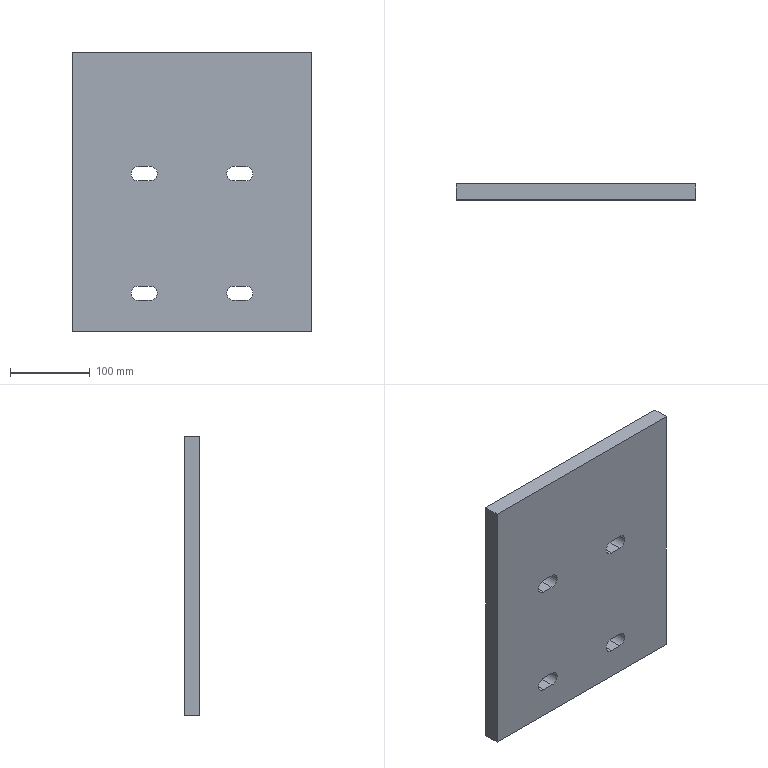Component | SolidWorks | WeldedI-beam-1_250I-beamMountingPlate-1 | 1 solid | 22 faces | box 300 x 20 x 350 mm | volume 2058042 mm3 | plane 14 | cylinder 8 | commonest cylinder face diameters 18 x8 | material Plain Carbon Steel
STEP:
#1=CARTESIAN_POINT('',(-256.79,105.58,213.545));
#2=VERTEX_POINT('',#1);
#3=CARTESIAN_POINT('',(-256.79,105.58,227.325));
#4=VERTEX_POINT('',#3);
#5=CARTESIAN_POINT('',(-256.79,105.58,213.545));
#6=DIRECTION('',(0.,0.,1.));
#7=VECTOR('',#6,39.37);
#8=LINE('',#5,#7);
#9=EDGE_CURVE('',#2,#4,#8,.T.);
#10=ORIENTED_EDGE('',*,*,#9,.F.);
#11=CARTESIAN_POINT('',(-256.79,104.793,213.545));
#12=VERTEX_POINT('',#11);
#13=CARTESIAN_POINT('',(-256.79,104.793,213.545));
#14=DIRECTION('',(0.,1.,0.));
#15=VECTOR('',#14,39.37);
#16=LINE('',#13,#15);
#17=EDGE_CURVE('',#12,#2,#16,.T.);
#18=ORIENTED_EDGE('',*,*,#17,.F.);
#19=CARTESIAN_POINT('',(-256.79,104.793,227.325));
#20=VERTEX_POINT('',#19);
#21=CARTESIAN_POINT('',(-256.79,104.793,213.545));
#22=DIRECTION('',(0.,0.,1.));
#23=VECTOR('',#22,39.37);
#24=LINE('',#21,#23);
#25=EDGE_CURVE('',#12,#20,#24,.T.);
#26=ORIENTED_EDGE('',*,*,#25,.T.);
#27=CARTESIAN_POINT('',(-256.79,104.793,227.325));
#28=DIRECTION('',(0.,1.,0.));
#29=VECTOR('',#28,39.37);
#30=LINE('',#27,#29);
#31=EDGE_CURVE('',#20,#4,#30,.T.);
#32=ORIENTED_EDGE('',*,*,#31,.T.);
#33=EDGE_LOOP('',(#10,#18,#26,#32));
#34=FACE_OUTER_BOUND('',#33,.T.);
#35=CARTESIAN_POINT('',(-256.79,104.793,213.545));
#36=DIRECTION('',(-1.,0.,0.));
#37=DIRECTION('',(0.,0.,1.));
#38=AXIS2_PLACEMENT_3D('',#35,#36,#37);
#39=PLANE('',#38);
#40=ADVANCED_FACE('',(#34),#39,.T.);
#41=CARTESIAN_POINT('',(-244.979,105.58,213.545));
#42=VERTEX_POINT('',#41);
#43=CARTESIAN_POINT('',(-256.79,105.58,213.545));
#44=DIRECTION('',(-1.,0.,0.));
#45=VECTOR('',#44,39.37);
#46=LINE('',#43,#45);
#47=EDGE_CURVE('',#42,#2,#46,.T.);
#48=ORIENTED_EDGE('',*,*,#47,.F.);
#49=CARTESIAN_POINT('',(-244.979,104.793,213.545));
#50=VERTEX_POINT('',#49);
#51=CARTESIAN_POINT('',(-244.979,104.793,213.545));
#52=DIRECTION('',(0.,1.,0.));
#53=VECTOR('',#52,39.37);
#54=LINE('',#51,#53);
#55=EDGE_CURVE('',#50,#42,#54,.T.);
#56=ORIENTED_EDGE('',*,*,#55,.F.);
#57=CARTESIAN_POINT('',(-256.79,104.793,213.545));
#58=DIRECTION('',(-1.,0.,0.));
#59=VECTOR('',#58,39.37);
#60=LINE('',#57,#59);
#61=EDGE_CURVE('',#50,#12,#60,.T.);
#62=ORIENTED_EDGE('',*,*,#61,.T.);
#63=ORIENTED_EDGE('',*,*,#17,.T.);
#64=EDGE_LOOP('',(#48,#56,#62,#63));
#65=FACE_OUTER_BOUND('',#64,.T.);
#66=CARTESIAN_POINT('',(-256.79,104.793,213.545));
#67=DIRECTION('',(0.,0.,-1.));
#68=DIRECTION('',(-1.,0.,0.));
#69=AXIS2_PLACEMENT_3D('',#66,#67,#68);
#70=PLANE('',#69);
#71=ADVANCED_FACE('',(#65),#70,.T.);
#72=CARTESIAN_POINT('',(-244.979,105.58,227.325));
#73=VERTEX_POINT('',#72);
#74=CARTESIAN_POINT('',(-244.979,105.58,213.545));
#75=DIRECTION('',(-0.,0.,-1.));
#76=VECTOR('',#75,39.37);
#77=LINE('',#74,#76);
#78=EDGE_CURVE('',#73,#42,#77,.T.);
#79=ORIENTED_EDGE('',*,*,#78,.F.);
#80=CARTESIAN_POINT('',(-244.979,104.793,227.325));
#81=VERTEX_POINT('',#80);
#82=CARTESIAN_POINT('',(-244.979,104.793,227.325));
#83=DIRECTION('',(0.,1.,0.));
#84=VECTOR('',#83,39.37);
#85=LINE('',#82,#84);
#86=EDGE_CURVE('',#81,#73,#85,.T.);
#87=ORIENTED_EDGE('',*,*,#86,.F.);
#88=CARTESIAN_POINT('',(-244.979,104.793,213.545));
#89=DIRECTION('',(-0.,0.,-1.));
#90=VECTOR('',#89,39.37);
#91=LINE('',#88,#90);
#92=EDGE_CURVE('',#81,#50,#91,.T.);
#93=ORIENTED_EDGE('',*,*,#92,.T.);
#94=ORIENTED_EDGE('',*,*,#55,.T.);
#95=EDGE_LOOP('',(#79,#87,#93,#94));
#96=FACE_OUTER_BOUND('',#95,.T.);
#97=CARTESIAN_POINT('',(-244.979,104.793,213.545));
#98=DIRECTION('',(1.,0.,-0.));
#99=DIRECTION('',(-0.,0.,-1.));
#100=AXIS2_PLACEMENT_3D('',#97,#98,#99);
#101=PLANE('',#100);
#102=ADVANCED_FACE('',(#96),#101,.T.);
#103=CARTESIAN_POINT('',(-256.79,105.58,227.325));
#104=DIRECTION('',(1.,0.,0.));
#105=VECTOR('',#104,39.37);
#106=LINE('',#103,#105);
#107=EDGE_CURVE('',#4,#73,#106,.T.);
#108=ORIENTED_EDGE('',*,*,#107,.F.);
#109=ORIENTED_EDGE('',*,*,#31,.F.);
#110=CARTESIAN_POINT('',(-256.79,104.793,227.325));
#111=DIRECTION('',(1.,0.,0.));
#112=VECTOR('',#111,39.37);
#113=LINE('',#110,#112);
#114=EDGE_CURVE('',#20,#81,#113,.T.);
#115=ORIENTED_EDGE('',*,*,#114,.T.);
#116=ORIENTED_EDGE('',*,*,#86,.T.);
#117=EDGE_LOOP('',(#108,#109,#115,#116));
#118=FACE_OUTER_BOUND('',#117,.T.);
#119=CARTESIAN_POINT('',(-256.79,104.793,227.325));
#120=DIRECTION('',(0.,0.,1.));
#121=DIRECTION('',(1.,0.,0.));
#122=AXIS2_PLACEMENT_3D('',#119,#120,#121);
#123=PLANE('',#122);
#124=ADVANCED_FACE('',(#118),#123,.T.);
#125=CARTESIAN_POINT('',(-252.951,104.793,220.986));
#126=VERTEX_POINT('',#125);
#127=CARTESIAN_POINT('',(-253.542,104.793,220.986));
#128=VERTEX_POINT('',#127);
#129=CARTESIAN_POINT('',(-253.542,104.793,220.986));
#130=DIRECTION('',(-1.,0.,0.));
#131=VECTOR('',#130,39.37);
#132=LINE('',#129,#131);
#133=EDGE_CURVE('',#126,#128,#132,.T.);
#134=ORIENTED_EDGE('',*,*,#133,.T.);
#135=CARTESIAN_POINT('',(-253.542,104.793,221.695));
#136=VERTEX_POINT('',#135);
#137=CARTESIAN_POINT('',(-253.542,104.793,221.34));
#138=DIRECTION('',(0.,1.,0.));
#139=DIRECTION('',(0.,0.,1.));
#140=AXIS2_PLACEMENT_3D('',#137,#138,#139);
#141=CIRCLE('',#140,0.3543);
#142=EDGE_CURVE('',#128,#136,#141,.T.);
#143=ORIENTED_EDGE('',*,*,#142,.T.);
#144=CARTESIAN_POINT('',(-252.951,104.793,221.695));
#145=VERTEX_POINT('',#144);
#146=CARTESIAN_POINT('',(-253.542,104.793,221.695));
#147=DIRECTION('',(1.,0.,0.));
#148=VECTOR('',#147,39.37);
#149=LINE('',#146,#148);
#150=EDGE_CURVE('',#136,#145,#149,.T.);
#151=ORIENTED_EDGE('',*,*,#150,.T.);
#152=CARTESIAN_POINT('',(-252.951,104.793,221.34));
#153=DIRECTION('',(0.,1.,0.));
#154=DIRECTION('',(0.,0.,1.));
#155=AXIS2_PLACEMENT_3D('',#152,#153,#154);
#156=CIRCLE('',#155,0.3543);
#157=EDGE_CURVE('',#145,#126,#156,.T.);
#158=ORIENTED_EDGE('',*,*,#157,.T.);
#159=EDGE_LOOP('',(#134,#143,#151,#158));
#160=FACE_BOUND('',#159,.T.);
#161=CARTESIAN_POINT('',(-248.227,104.793,220.986));
#162=VERTEX_POINT('',#161);
#163=CARTESIAN_POINT('',(-248.818,104.793,220.986));
#164=VERTEX_POINT('',#163);
#165=CARTESIAN_POINT('',(-248.818,104.793,220.986));
#166=DIRECTION('',(-1.,0.,-0.));
#167=VECTOR('',#166,39.37);
#168=LINE('',#165,#167);
#169=EDGE_CURVE('',#162,#164,#168,.T.);
#170=ORIENTED_EDGE('',*,*,#169,.T.);
#171=CARTESIAN_POINT('',(-248.818,104.793,221.695));
#172=VERTEX_POINT('',#171);
#173=CARTESIAN_POINT('',(-248.818,104.793,221.34));
#174=DIRECTION('',(0.,1.,0.));
#175=DIRECTION('',(0.,0.,1.));
#176=AXIS2_PLACEMENT_3D('',#173,#174,#175);
#177=CIRCLE('',#176,0.3543);
#178=EDGE_CURVE('',#164,#172,#177,.T.);
#179=ORIENTED_EDGE('',*,*,#178,.T.);
#180=CARTESIAN_POINT('',(-248.227,104.793,221.695));
#181=VERTEX_POINT('',#180);
#182=CARTESIAN_POINT('',(-248.818,104.793,221.695));
#183=DIRECTION('',(1.,0.,-0.));
#184=VECTOR('',#183,39.37);
#185=LINE('',#182,#184);
#186=EDGE_CURVE('',#172,#181,#185,.T.);
#187=ORIENTED_EDGE('',*,*,#186,.T.);
#188=CARTESIAN_POINT('',(-248.227,104.793,221.34));
#189=DIRECTION('',(0.,1.,0.));
#190=DIRECTION('',(0.,0.,1.));
#191=AXIS2_PLACEMENT_3D('',#188,#189,#190);
#192=CIRCLE('',#191,0.3543);
#193=EDGE_CURVE('',#181,#162,#192,.T.);
#194=ORIENTED_EDGE('',*,*,#193,.T.);
#195=EDGE_LOOP('',(#170,#179,#187,#194));
#196=FACE_BOUND('',#195,.T.);
#197=CARTESIAN_POINT('',(-252.951,104.793,215.08));
#198=VERTEX_POINT('',#197);
#199=CARTESIAN_POINT('',(-253.542,104.793,215.08));
#200=VERTEX_POINT('',#199);
#201=CARTESIAN_POINT('',(-253.542,104.793,215.08));
#202=DIRECTION('',(-1.,0.,0.));
#203=VECTOR('',#202,39.37);
#204=LINE('',#201,#203);
#205=EDGE_CURVE('',#198,#200,#204,.T.);
#206=ORIENTED_EDGE('',*,*,#205,.T.);
#207=CARTESIAN_POINT('',(-253.542,104.793,215.789));
#208=VERTEX_POINT('',#207);
#209=CARTESIAN_POINT('',(-253.542,104.793,215.435));
#210=DIRECTION('',(0.,1.,0.));
#211=DIRECTION('',(0.,0.,1.));
#212=AXIS2_PLACEMENT_3D('',#209,#210,#211);
#213=CIRCLE('',#212,0.3543);
#214=EDGE_CURVE('',#200,#208,#213,.T.);
#215=ORIENTED_EDGE('',*,*,#214,.T.);
#216=CARTESIAN_POINT('',(-252.951,104.793,215.789));
#217=VERTEX_POINT('',#216);
#218=CARTESIAN_POINT('',(-253.542,104.793,215.789));
#219=DIRECTION('',(1.,0.,0.));
#220=VECTOR('',#219,39.37);
#221=LINE('',#218,#220);
#222=EDGE_CURVE('',#208,#217,#221,.T.);
#223=ORIENTED_EDGE('',*,*,#222,.T.);
#224=CARTESIAN_POINT('',(-252.951,104.793,215.435));
#225=DIRECTION('',(0.,1.,0.));
#226=DIRECTION('',(0.,0.,1.));
#227=AXIS2_PLACEMENT_3D('',#224,#225,#226);
#228=CIRCLE('',#227,0.3543);
#229=EDGE_CURVE('',#217,#198,#228,.T.);
#230=ORIENTED_EDGE('',*,*,#229,.T.);
#231=EDGE_LOOP('',(#206,#215,#223,#230));
#232=FACE_BOUND('',#231,.T.);
#233=CARTESIAN_POINT('',(-248.227,104.793,215.08));
#234=VERTEX_POINT('',#233);
#235=CARTESIAN_POINT('',(-248.818,104.793,215.08));
#236=VERTEX_POINT('',#235);
#237=CARTESIAN_POINT('',(-248.818,104.793,215.08));
#238=DIRECTION('',(-1.,0.,0.));
#239=VECTOR('',#238,39.37);
#240=LINE('',#237,#239);
#241=EDGE_CURVE('',#234,#236,#240,.T.);
#242=ORIENTED_EDGE('',*,*,#241,.T.);
#243=CARTESIAN_POINT('',(-248.818,104.793,215.789));
#244=VERTEX_POINT('',#243);
#245=CARTESIAN_POINT('',(-248.818,104.793,215.435));
#246=DIRECTION('',(0.,1.,0.));
#247=DIRECTION('',(0.,0.,1.));
#248=AXIS2_PLACEMENT_3D('',#245,#246,#247);
#249=CIRCLE('',#248,0.3543);
#250=EDGE_CURVE('',#236,#244,#249,.T.);
#251=ORIENTED_EDGE('',*,*,#250,.T.);
#252=CARTESIAN_POINT('',(-248.227,104.793,215.789));
#253=VERTEX_POINT('',#252);
#254=CARTESIAN_POINT('',(-248.818,104.793,215.789));
#255=DIRECTION('',(1.,0.,0.));
#256=VECTOR('',#255,39.37);
#257=LINE('',#254,#256);
#258=EDGE_CURVE('',#244,#253,#257,.T.);
#259=ORIENTED_EDGE('',*,*,#258,.T.);
#260=CARTESIAN_POINT('',(-248.227,104.793,215.435));
#261=DIRECTION('',(0.,1.,0.));
#262=DIRECTION('',(0.,0.,1.));
#263=AXIS2_PLACEMENT_3D('',#260,#261,#262);
#264=CIRCLE('',#263,0.3543);
#265=EDGE_CURVE('',#253,#234,#264,.T.);
#266=ORIENTED_EDGE('',*,*,#265,.T.);
#267=EDGE_LOOP('',(#242,#251,#259,#266));
#268=FACE_BOUND('',#267,.T.);
#269=ORIENTED_EDGE('',*,*,#25,.F.);
#270=ORIENTED_EDGE('',*,*,#61,.F.);
#271=ORIENTED_EDGE('',*,*,#92,.F.);
#272=ORIENTED_EDGE('',*,*,#114,.F.);
#273=EDGE_LOOP('',(#269,#270,#271,#272));
#274=FACE_OUTER_BOUND('',#273,.T.);
#275=CARTESIAN_POINT('',(-256.79,104.793,213.545));
#276=DIRECTION('',(0.,1.,0.));
#277=DIRECTION('',(0.,0.,1.));
#278=AXIS2_PLACEMENT_3D('',#275,#276,#277);
#279=PLANE('',#278);
#280=ADVANCED_FACE('',(#160,#196,#232,#268,#274),#279,.F.);
#281=CARTESIAN_POINT('',(-253.542,105.58,220.986));
#282=VERTEX_POINT('',#281);
#283=CARTESIAN_POINT('',(-253.542,105.58,221.695));
#284=VERTEX_POINT('',#283);
#285=CARTESIAN_POINT('',(-253.542,105.58,221.34));
#286=DIRECTION('',(0.,1.,0.));
#287=DIRECTION('',(0.,0.,1.));
#288=AXIS2_PLACEMENT_3D('',#285,#286,#287);
#289=CIRCLE('',#288,0.3543);
#290=EDGE_CURVE('',#282,#284,#289,.T.);
#291=ORIENTED_EDGE('',*,*,#290,.F.);
#292=CARTESIAN_POINT('',(-252.951,105.58,220.986));
#293=VERTEX_POINT('',#292);
#294=CARTESIAN_POINT('',(-253.542,105.58,220.986));
#295=DIRECTION('',(-1.,0.,0.));
#296=VECTOR('',#295,39.37);
#297=LINE('',#294,#296);
#298=EDGE_CURVE('',#293,#282,#297,.T.);
#299=ORIENTED_EDGE('',*,*,#298,.F.);
#300=CARTESIAN_POINT('',(-252.951,105.58,221.695));
#301=VERTEX_POINT('',#300);
#302=CARTESIAN_POINT('',(-252.951,105.58,221.34));
#303=DIRECTION('',(0.,1.,0.));
#304=DIRECTION('',(0.,0.,1.));
#305=AXIS2_PLACEMENT_3D('',#302,#303,#304);
#306=CIRCLE('',#305,0.3543);
#307=EDGE_CURVE('',#301,#293,#306,.T.);
#308=ORIENTED_EDGE('',*,*,#307,.F.);
#309=CARTESIAN_POINT('',(-253.542,105.58,221.695));
#310=DIRECTION('',(1.,0.,0.));
#311=VECTOR('',#310,39.37);
#312=LINE('',#309,#311);
#313=EDGE_CURVE('',#284,#301,#312,.T.);
#314=ORIENTED_EDGE('',*,*,#313,.F.);
#315=EDGE_LOOP('',(#291,#299,#308,#314));
#316=FACE_BOUND('',#315,.T.);
#317=CARTESIAN_POINT('',(-248.818,105.58,220.986));
#318=VERTEX_POINT('',#317);
#319=CARTESIAN_POINT('',(-248.818,105.58,221.695));
#320=VERTEX_POINT('',#319);
#321=CARTESIAN_POINT('',(-248.818,105.58,221.34));
#322=DIRECTION('',(0.,1.,0.));
#323=DIRECTION('',(0.,0.,1.));
#324=AXIS2_PLACEMENT_3D('',#321,#322,#323);
#325=CIRCLE('',#324,0.3543);
#326=EDGE_CURVE('',#318,#320,#325,.T.);
#327=ORIENTED_EDGE('',*,*,#326,.F.);
#328=CARTESIAN_POINT('',(-248.227,105.58,220.986));
#329=VERTEX_POINT('',#328);
#330=CARTESIAN_POINT('',(-248.818,105.58,220.986));
#331=DIRECTION('',(-1.,0.,-0.));
#332=VECTOR('',#331,39.37);
#333=LINE('',#330,#332);
#334=EDGE_CURVE('',#329,#318,#333,.T.);
#335=ORIENTED_EDGE('',*,*,#334,.F.);
#336=CARTESIAN_POINT('',(-248.227,105.58,221.695));
#337=VERTEX_POINT('',#336);
#338=CARTESIAN_POINT('',(-248.227,105.58,221.34));
#339=DIRECTION('',(0.,1.,0.));
#340=DIRECTION('',(0.,0.,1.));
#341=AXIS2_PLACEMENT_3D('',#338,#339,#340);
#342=CIRCLE('',#341,0.3543);
#343=EDGE_CURVE('',#337,#329,#342,.T.);
#344=ORIENTED_EDGE('',*,*,#343,.F.);
#345=CARTESIAN_POINT('',(-248.818,105.58,221.695));
#346=DIRECTION('',(1.,0.,-0.));
#347=VECTOR('',#346,39.37);
#348=LINE('',#345,#347);
#349=EDGE_CURVE('',#320,#337,#348,.T.);
#350=ORIENTED_EDGE('',*,*,#349,.F.);
#351=EDGE_LOOP('',(#327,#335,#344,#350));
#352=FACE_BOUND('',#351,.T.);
#353=CARTESIAN_POINT('',(-253.542,105.58,215.08));
#354=VERTEX_POINT('',#353);
#355=CARTESIAN_POINT('',(-253.542,105.58,215.789));
#356=VERTEX_POINT('',#355);
#357=CARTESIAN_POINT('',(-253.542,105.58,215.435));
#358=DIRECTION('',(0.,1.,0.));
#359=DIRECTION('',(0.,0.,1.));
#360=AXIS2_PLACEMENT_3D('',#357,#358,#359);
#361=CIRCLE('',#360,0.3543);
#362=EDGE_CURVE('',#354,#356,#361,.T.);
#363=ORIENTED_EDGE('',*,*,#362,.F.);
#364=CARTESIAN_POINT('',(-252.951,105.58,215.08));
#365=VERTEX_POINT('',#364);
#366=CARTESIAN_POINT('',(-253.542,105.58,215.08));
#367=DIRECTION('',(-1.,0.,0.));
#368=VECTOR('',#367,39.37);
#369=LINE('',#366,#368);
#370=EDGE_CURVE('',#365,#354,#369,.T.);
#371=ORIENTED_EDGE('',*,*,#370,.F.);
#372=CARTESIAN_POINT('',(-252.951,105.58,215.789));
#373=VERTEX_POINT('',#372);
#374=CARTESIAN_POINT('',(-252.951,105.58,215.435));
#375=DIRECTION('',(0.,1.,0.));
#376=DIRECTION('',(0.,0.,1.));
#377=AXIS2_PLACEMENT_3D('',#374,#375,#376);
#378=CIRCLE('',#377,0.3543);
#379=EDGE_CURVE('',#373,#365,#378,.T.);
#380=ORIENTED_EDGE('',*,*,#379,.F.);
#381=CARTESIAN_POINT('',(-253.542,105.58,215.789));
#382=DIRECTION('',(1.,0.,0.));
#383=VECTOR('',#382,39.37);
#384=LINE('',#381,#383);
#385=EDGE_CURVE('',#356,#373,#384,.T.);
#386=ORIENTED_EDGE('',*,*,#385,.F.);
#387=EDGE_LOOP('',(#363,#371,#380,#386));
#388=FACE_BOUND('',#387,.T.);
#389=CARTESIAN_POINT('',(-248.818,105.58,215.08));
#390=VERTEX_POINT('',#389);
#391=CARTESIAN_POINT('',(-248.818,105.58,215.789));
#392=VERTEX_POINT('',#391);
#393=CARTESIAN_POINT('',(-248.818,105.58,215.435));
#394=DIRECTION('',(0.,1.,0.));
#395=DIRECTION('',(0.,0.,1.));
#396=AXIS2_PLACEMENT_3D('',#393,#394,#395);
#397=CIRCLE('',#396,0.3543);
#398=EDGE_CURVE('',#390,#392,#397,.T.);
#399=ORIENTED_EDGE('',*,*,#398,.F.);
#400=CARTESIAN_POINT('',(-248.227,105.58,215.08));
#401=VERTEX_POINT('',#400);
#402=CARTESIAN_POINT('',(-248.818,105.58,215.08));
#403=DIRECTION('',(-1.,0.,0.));
#404=VECTOR('',#403,39.37);
#405=LINE('',#402,#404);
#406=EDGE_CURVE('',#401,#390,#405,.T.);
#407=ORIENTED_EDGE('',*,*,#406,.F.);
#408=CARTESIAN_POINT('',(-248.227,105.58,215.789));
#409=VERTEX_POINT('',#408);
#410=CARTESIAN_POINT('',(-248.227,105.58,215.435));
#411=DIRECTION('',(0.,1.,0.));
#412=DIRECTION('',(0.,0.,1.));
#413=AXIS2_PLACEMENT_3D('',#410,#411,#412);
#414=CIRCLE('',#413,0.3543);
#415=EDGE_CURVE('',#409,#401,#414,.T.);
#416=ORIENTED_EDGE('',*,*,#415,.F.);
#417=CARTESIAN_POINT('',(-248.818,105.58,215.789));
#418=DIRECTION('',(1.,0.,0.));
#419=VECTOR('',#418,39.37);
#420=LINE('',#417,#419);
#421=EDGE_CURVE('',#392,#409,#420,.T.);
#422=ORIENTED_EDGE('',*,*,#421,.F.);
#423=EDGE_LOOP('',(#399,#407,#416,#422));
#424=FACE_BOUND('',#423,.T.);
#425=ORIENTED_EDGE('',*,*,#9,.T.);
#426=ORIENTED_EDGE('',*,*,#107,.T.);
#427=ORIENTED_EDGE('',*,*,#78,.T.);
#428=ORIENTED_EDGE('',*,*,#47,.T.);
#429=EDGE_LOOP('',(#425,#426,#427,#428));
#430=FACE_OUTER_BOUND('',#429,.T.);
#431=CARTESIAN_POINT('',(-256.79,105.58,213.545));
#432=DIRECTION('',(0.,1.,0.));
#433=DIRECTION('',(0.,0.,1.));
#434=AXIS2_PLACEMENT_3D('',#431,#432,#433);
#435=PLANE('',#434);
#436=ADVANCED_FACE('',(#316,#352,#388,#424,#430),#435,.T.);
#437=ORIENTED_EDGE('',*,*,#398,.T.);
#438=CARTESIAN_POINT('',(-248.818,104.793,215.789));
#439=DIRECTION('',(0.,1.,0.));
#440=VECTOR('',#439,39.37);
#441=LINE('',#438,#440);
#442=EDGE_CURVE('',#244,#392,#441,.T.);
#443=ORIENTED_EDGE('',*,*,#442,.F.);
#444=ORIENTED_EDGE('',*,*,#250,.F.);
#445=CARTESIAN_POINT('',(-248.818,104.793,215.08));
#446=DIRECTION('',(0.,1.,0.));
#447=VECTOR('',#446,39.37);
#448=LINE('',#445,#447);
#449=EDGE_CURVE('',#236,#390,#448,.T.);
#450=ORIENTED_EDGE('',*,*,#449,.T.);
#451=EDGE_LOOP('',(#437,#443,#444,#450));
#452=FACE_OUTER_BOUND('',#451,.T.);
#453=CARTESIAN_POINT('',(-248.818,104.793,215.435));
#454=DIRECTION('',(0.,1.,0.));
#455=DIRECTION('',(0.,0.,1.));
#456=AXIS2_PLACEMENT_3D('',#453,#454,#455);
#457=CYLINDRICAL_SURFACE('',#456,0.3543);
#458=ADVANCED_FACE('',(#452),#457,.F.);
#459=ORIENTED_EDGE('',*,*,#406,.T.);
#460=ORIENTED_EDGE('',*,*,#449,.F.);
#461=ORIENTED_EDGE('',*,*,#241,.F.);
#462=CARTESIAN_POINT('',(-248.227,104.793,215.08));
#463=DIRECTION('',(0.,1.,0.));
#464=VECTOR('',#463,39.37);
#465=LINE('',#462,#464);
#466=EDGE_CURVE('',#234,#401,#465,.T.);
#467=ORIENTED_EDGE('',*,*,#466,.T.);
#468=EDGE_LOOP('',(#459,#460,#461,#467));
#469=FACE_OUTER_BOUND('',#468,.T.);
#470=CARTESIAN_POINT('',(-248.818,104.793,215.08));
#471=DIRECTION('',(0.,0.,-1.));
#472=DIRECTION('',(-1.,0.,0.));
#473=AXIS2_PLACEMENT_3D('',#470,#471,#472);
#474=PLANE('',#473);
#475=ADVANCED_FACE('',(#469),#474,.F.);
#476=ORIENTED_EDGE('',*,*,#415,.T.);
#477=ORIENTED_EDGE('',*,*,#466,.F.);
#478=ORIENTED_EDGE('',*,*,#265,.F.);
#479=CARTESIAN_POINT('',(-248.227,104.793,215.789));
#480=DIRECTION('',(0.,1.,0.));
#481=VECTOR('',#480,39.37);
#482=LINE('',#479,#481);
#483=EDGE_CURVE('',#253,#409,#482,.T.);
#484=ORIENTED_EDGE('',*,*,#483,.T.);
#485=EDGE_LOOP('',(#476,#477,#478,#484));
#486=FACE_OUTER_BOUND('',#485,.T.);
#487=CARTESIAN_POINT('',(-248.227,104.793,215.435));
#488=DIRECTION('',(0.,1.,0.));
#489=DIRECTION('',(0.,0.,1.));
#490=AXIS2_PLACEMENT_3D('',#487,#488,#489);
#491=CYLINDRICAL_SURFACE('',#490,0.3543);
#492=ADVANCED_FACE('',(#486),#491,.F.);
#493=ORIENTED_EDGE('',*,*,#421,.T.);
#494=ORIENTED_EDGE('',*,*,#483,.F.);
#495=ORIENTED_EDGE('',*,*,#258,.F.);
#496=ORIENTED_EDGE('',*,*,#442,.T.);
#497=EDGE_LOOP('',(#493,#494,#495,#496));
#498=FACE_OUTER_BOUND('',#497,.T.);
#499=CARTESIAN_POINT('',(-248.818,104.793,215.789));
#500=DIRECTION('',(0.,0.,1.));
#501=DIRECTION('',(1.,0.,0.));
#502=AXIS2_PLACEMENT_3D('',#499,#500,#501);
#503=PLANE('',#502);
#504=ADVANCED_FACE('',(#498),#503,.F.);
#505=ORIENTED_EDGE('',*,*,#362,.T.);
#506=CARTESIAN_POINT('',(-253.542,104.793,215.789));
#507=DIRECTION('',(0.,1.,0.));
#508=VECTOR('',#507,39.37);
#509=LINE('',#506,#508);
#510=EDGE_CURVE('',#208,#356,#509,.T.);
#511=ORIENTED_EDGE('',*,*,#510,.F.);
#512=ORIENTED_EDGE('',*,*,#214,.F.);
#513=CARTESIAN_POINT('',(-253.542,104.793,215.08));
#514=DIRECTION('',(0.,1.,0.));
#515=VECTOR('',#514,39.37);
#516=LINE('',#513,#515);
#517=EDGE_CURVE('',#200,#354,#516,.T.);
#518=ORIENTED_EDGE('',*,*,#517,.T.);
#519=EDGE_LOOP('',(#505,#511,#512,#518));
#520=FACE_OUTER_BOUND('',#519,.T.);
#521=CARTESIAN_POINT('',(-253.542,104.793,215.435));
#522=DIRECTION('',(0.,1.,0.));
#523=DIRECTION('',(0.,0.,1.));
#524=AXIS2_PLACEMENT_3D('',#521,#522,#523);
#525=CYLINDRICAL_SURFACE('',#524,0.3543);
#526=ADVANCED_FACE('',(#520),#525,.F.);
#527=ORIENTED_EDGE('',*,*,#370,.T.);
#528=ORIENTED_EDGE('',*,*,#517,.F.);
#529=ORIENTED_EDGE('',*,*,#205,.F.);
#530=CARTESIAN_POINT('',(-252.951,104.793,215.08));
#531=DIRECTION('',(0.,1.,0.));
#532=VECTOR('',#531,39.37);
#533=LINE('',#530,#532);
#534=EDGE_CURVE('',#198,#365,#533,.T.);
#535=ORIENTED_EDGE('',*,*,#534,.T.);
#536=EDGE_LOOP('',(#527,#528,#529,#535));
#537=FACE_OUTER_BOUND('',#536,.T.);
#538=CARTESIAN_POINT('',(-253.542,104.793,215.08));
#539=DIRECTION('',(0.,0.,-1.));
#540=DIRECTION('',(-1.,0.,0.));
#541=AXIS2_PLACEMENT_3D('',#538,#539,#540);
#542=PLANE('',#541);
#543=ADVANCED_FACE('',(#537),#542,.F.);
#544=ORIENTED_EDGE('',*,*,#379,.T.);
#545=ORIENTED_EDGE('',*,*,#534,.F.);
#546=ORIENTED_EDGE('',*,*,#229,.F.);
#547=CARTESIAN_POINT('',(-252.951,104.793,215.789));
#548=DIRECTION('',(0.,1.,0.));
#549=VECTOR('',#548,39.37);
#550=LINE('',#547,#549);
#551=EDGE_CURVE('',#217,#373,#550,.T.);
#552=ORIENTED_EDGE('',*,*,#551,.T.);
#553=EDGE_LOOP('',(#544,#545,#546,#552));
#554=FACE_OUTER_BOUND('',#553,.T.);
#555=CARTESIAN_POINT('',(-252.951,104.793,215.435));
#556=DIRECTION('',(0.,1.,0.));
#557=DIRECTION('',(0.,0.,1.));
#558=AXIS2_PLACEMENT_3D('',#555,#556,#557);
#559=CYLINDRICAL_SURFACE('',#558,0.3543);
#560=ADVANCED_FACE('',(#554),#559,.F.);
#561=ORIENTED_EDGE('',*,*,#385,.T.);
#562=ORIENTED_EDGE('',*,*,#551,.F.);
#563=ORIENTED_EDGE('',*,*,#222,.F.);
#564=ORIENTED_EDGE('',*,*,#510,.T.);
#565=EDGE_LOOP('',(#561,#562,#563,#564));
#566=FACE_OUTER_BOUND('',#565,.T.);
#567=CARTESIAN_POINT('',(-253.542,104.793,215.789));
#568=DIRECTION('',(0.,0.,1.));
#569=DIRECTION('',(1.,0.,0.));
#570=AXIS2_PLACEMENT_3D('',#567,#568,#569);
#571=PLANE('',#570);
#572=ADVANCED_FACE('',(#566),#571,.F.);
#573=ORIENTED_EDGE('',*,*,#326,.T.);
#574=CARTESIAN_POINT('',(-248.818,104.793,221.695));
#575=DIRECTION('',(0.,1.,0.));
#576=VECTOR('',#575,39.37);
#577=LINE('',#574,#576);
#578=EDGE_CURVE('',#172,#320,#577,.T.);
#579=ORIENTED_EDGE('',*,*,#578,.F.);
#580=ORIENTED_EDGE('',*,*,#178,.F.);
#581=CARTESIAN_POINT('',(-248.818,104.793,220.986));
#582=DIRECTION('',(0.,1.,0.));
#583=VECTOR('',#582,39.37);
#584=LINE('',#581,#583);
#585=EDGE_CURVE('',#164,#318,#584,.T.);
#586=ORIENTED_EDGE('',*,*,#585,.T.);
#587=EDGE_LOOP('',(#573,#579,#580,#586));
#588=FACE_OUTER_BOUND('',#587,.T.);
#589=CARTESIAN_POINT('',(-248.818,104.793,221.34));
#590=DIRECTION('',(0.,1.,0.));
#591=DIRECTION('',(0.,0.,1.));
#592=AXIS2_PLACEMENT_3D('',#589,#590,#591);
#593=CYLINDRICAL_SURFACE('',#592,0.3543);
#594=ADVANCED_FACE('',(#588),#593,.F.);
#595=ORIENTED_EDGE('',*,*,#334,.T.);
#596=ORIENTED_EDGE('',*,*,#585,.F.);
#597=ORIENTED_EDGE('',*,*,#169,.F.);
#598=CARTESIAN_POINT('',(-248.227,104.793,220.986));
#599=DIRECTION('',(0.,1.,0.));
#600=VECTOR('',#599,39.37);
#601=LINE('',#598,#600);
#602=EDGE_CURVE('',#162,#329,#601,.T.);
#603=ORIENTED_EDGE('',*,*,#602,.T.);
#604=EDGE_LOOP('',(#595,#596,#597,#603));
#605=FACE_OUTER_BOUND('',#604,.T.);
#606=CARTESIAN_POINT('',(-248.818,104.793,220.986));
#607=DIRECTION('',(0.,0.,-1.));
#608=DIRECTION('',(-1.,0.,-0.));
#609=AXIS2_PLACEMENT_3D('',#606,#607,#608);
#610=PLANE('',#609);
#611=ADVANCED_FACE('',(#605),#610,.F.);
#612=ORIENTED_EDGE('',*,*,#343,.T.);
#613=ORIENTED_EDGE('',*,*,#602,.F.);
#614=ORIENTED_EDGE('',*,*,#193,.F.);
#615=CARTESIAN_POINT('',(-248.227,104.793,221.695));
#616=DIRECTION('',(0.,1.,0.));
#617=VECTOR('',#616,39.37);
#618=LINE('',#615,#617);
#619=EDGE_CURVE('',#181,#337,#618,.T.);
#620=ORIENTED_EDGE('',*,*,#619,.T.);
#621=EDGE_LOOP('',(#612,#613,#614,#620));
#622=FACE_OUTER_BOUND('',#621,.T.);
#623=CARTESIAN_POINT('',(-248.227,104.793,221.34));
#624=DIRECTION('',(0.,1.,0.));
#625=DIRECTION('',(0.,0.,1.));
#626=AXIS2_PLACEMENT_3D('',#623,#624,#625);
#627=CYLINDRICAL_SURFACE('',#626,0.3543);
#628=ADVANCED_FACE('',(#622),#627,.F.);
#629=ORIENTED_EDGE('',*,*,#349,.T.);
#630=ORIENTED_EDGE('',*,*,#619,.F.);
#631=ORIENTED_EDGE('',*,*,#186,.F.);
#632=ORIENTED_EDGE('',*,*,#578,.T.);
#633=EDGE_LOOP('',(#629,#630,#631,#632));
#634=FACE_OUTER_BOUND('',#633,.T.);
#635=CARTESIAN_POINT('',(-248.818,104.793,221.695));
#636=DIRECTION('',(0.,0.,1.));
#637=DIRECTION('',(1.,0.,-0.));
#638=AXIS2_PLACEMENT_3D('',#635,#636,#637);
#639=PLANE('',#638);
#640=ADVANCED_FACE('',(#634),#639,.F.);
#641=ORIENTED_EDGE('',*,*,#290,.T.);
#642=CARTESIAN_POINT('',(-253.542,104.793,221.695));
#643=DIRECTION('',(0.,1.,0.));
#644=VECTOR('',#643,39.37);
#645=LINE('',#642,#644);
#646=EDGE_CURVE('',#136,#284,#645,.T.);
#647=ORIENTED_EDGE('',*,*,#646,.F.);
#648=ORIENTED_EDGE('',*,*,#142,.F.);
#649=CARTESIAN_POINT('',(-253.542,104.793,220.986));
#650=DIRECTION('',(0.,1.,0.));
#651=VECTOR('',#650,39.37);
#652=LINE('',#649,#651);
#653=EDGE_CURVE('',#128,#282,#652,.T.);
#654=ORIENTED_EDGE('',*,*,#653,.T.);
#655=EDGE_LOOP('',(#641,#647,#648,#654));
#656=FACE_OUTER_BOUND('',#655,.T.);
#657=CARTESIAN_POINT('',(-253.542,104.793,221.34));
#658=DIRECTION('',(0.,1.,0.));
#659=DIRECTION('',(0.,0.,1.));
#660=AXIS2_PLACEMENT_3D('',#657,#658,#659);
#661=CYLINDRICAL_SURFACE('',#660,0.3543);
#662=ADVANCED_FACE('',(#656),#661,.F.);
#663=ORIENTED_EDGE('',*,*,#298,.T.);
#664=ORIENTED_EDGE('',*,*,#653,.F.);
#665=ORIENTED_EDGE('',*,*,#133,.F.);
#666=CARTESIAN_POINT('',(-252.951,104.793,220.986));
#667=DIRECTION('',(0.,1.,0.));
#668=VECTOR('',#667,39.37);
#669=LINE('',#666,#668);
#670=EDGE_CURVE('',#126,#293,#669,.T.);
#671=ORIENTED_EDGE('',*,*,#670,.T.);
#672=EDGE_LOOP('',(#663,#664,#665,#671));
#673=FACE_OUTER_BOUND('',#672,.T.);
#674=CARTESIAN_POINT('',(-253.542,104.793,220.986));
#675=DIRECTION('',(0.,0.,-1.));
#676=DIRECTION('',(-1.,0.,0.));
#677=AXIS2_PLACEMENT_3D('',#674,#675,#676);
#678=PLANE('',#677);
#679=ADVANCED_FACE('',(#673),#678,.F.);
#680=ORIENTED_EDGE('',*,*,#307,.T.);
#681=ORIENTED_EDGE('',*,*,#670,.F.);
#682=ORIENTED_EDGE('',*,*,#157,.F.);
#683=CARTESIAN_POINT('',(-252.951,104.793,221.695));
#684=DIRECTION('',(0.,1.,0.));
#685=VECTOR('',#684,39.37);
#686=LINE('',#683,#685);
#687=EDGE_CURVE('',#145,#301,#686,.T.);
#688=ORIENTED_EDGE('',*,*,#687,.T.);
#689=EDGE_LOOP('',(#680,#681,#682,#688));
#690=FACE_OUTER_BOUND('',#689,.T.);
#691=CARTESIAN_POINT('',(-252.951,104.793,221.34));
#692=DIRECTION('',(0.,1.,0.));
#693=DIRECTION('',(0.,0.,1.));
#694=AXIS2_PLACEMENT_3D('',#691,#692,#693);
#695=CYLINDRICAL_SURFACE('',#694,0.3543);
#696=ADVANCED_FACE('',(#690),#695,.F.);
#697=ORIENTED_EDGE('',*,*,#313,.T.);
#698=ORIENTED_EDGE('',*,*,#687,.F.);
#699=ORIENTED_EDGE('',*,*,#150,.F.);
#700=ORIENTED_EDGE('',*,*,#646,.T.);
#701=EDGE_LOOP('',(#697,#698,#699,#700));
#702=FACE_OUTER_BOUND('',#701,.T.);
#703=CARTESIAN_POINT('',(-253.542,104.793,221.695));
#704=DIRECTION('',(0.,0.,1.));
#705=DIRECTION('',(1.,0.,0.));
#706=AXIS2_PLACEMENT_3D('',#703,#704,#705);
#707=PLANE('',#706);
#708=ADVANCED_FACE('',(#702),#707,.F.);
#709=CLOSED_SHELL('',(#40,#71,#102,#124,#280,#436,#458,#475,#492,#504,#526,#543,#560,#572,#594,#611,#628,#640,#662,#679,#696,#708));
#710=MANIFOLD_SOLID_BREP('',#709);
#711=CARTESIAN_POINT('',(0.,0.,0.));
#712=DIRECTION('',(0.,0.,1.));
#713=DIRECTION('',(1.,0.,0.));
#714=AXIS2_PLACEMENT_3D('',#711,#712,#713);
#715=(LENGTH_UNIT()NAMED_UNIT(*)SI_UNIT($,.METRE.));
#716=LENGTH_MEASURE_WITH_UNIT(LENGTH_MEASURE(0.0254),#715);
#717=DIMENSIONAL_EXPONENTS(1.,0.,0.,0.,0.,0.,0.);
#718=(CONVERSION_BASED_UNIT('',#716)LENGTH_UNIT()NAMED_UNIT(#717));
#719=UNCERTAINTY_MEASURE_WITH_UNIT(LENGTH_MEASURE(0.00001),#718,'','');
#720=(NAMED_UNIT(*)PLANE_ANGLE_UNIT()SI_UNIT($,.RADIAN.));
#721=(NAMED_UNIT(*)SI_UNIT($,.STERADIAN.)SOLID_ANGLE_UNIT());
#722=(GEOMETRIC_REPRESENTATION_CONTEXT(3)GLOBAL_UNCERTAINTY_ASSIGNED_CONTEXT((#719))GLOBAL_UNIT_ASSIGNED_CONTEXT((#718,#720,#721))REPRESENTATION_CONTEXT('',''));
#723=ADVANCED_BREP_SHAPE_REPRESENTATION('',(#710,#714),#722);
#724=COLOUR_RGB('',0.7922,0.8196,0.9333);
#725=FILL_AREA_STYLE_COLOUR('',#724);
#726=FILL_AREA_STYLE('',(#725));
#727=SURFACE_STYLE_FILL_AREA(#726);
#728=SURFACE_SIDE_STYLE('',(#727));
#729=SURFACE_STYLE_USAGE(.BOTH.,#728);
#730=PRESENTATION_STYLE_ASSIGNMENT((#729));
#731=STYLED_ITEM('',(#730),#710);
#732=PRESENTATION_LAYER_ASSIGNMENT('','',(#731));
#733=(LENGTH_UNIT()NAMED_UNIT(*)SI_UNIT($,.METRE.));
#734=LENGTH_MEASURE_WITH_UNIT(LENGTH_MEASURE(0.0254),#733);
#735=DIMENSIONAL_EXPONENTS(1.,0.,0.,0.,0.,0.,0.);
#736=(CONVERSION_BASED_UNIT('',#734)LENGTH_UNIT()NAMED_UNIT(#735));
#737=UNCERTAINTY_MEASURE_WITH_UNIT(LENGTH_MEASURE(0.00001),#736,'','');
#738=(NAMED_UNIT(*)PLANE_ANGLE_UNIT()SI_UNIT($,.RADIAN.));
#739=(NAMED_UNIT(*)SI_UNIT($,.STERADIAN.)SOLID_ANGLE_UNIT());
#740=(GEOMETRIC_REPRESENTATION_CONTEXT(3)GLOBAL_UNCERTAINTY_ASSIGNED_CONTEXT((#737))GLOBAL_UNIT_ASSIGNED_CONTEXT((#736,#738,#739))REPRESENTATION_CONTEXT('',''));
#741=MECHANICAL_DESIGN_GEOMETRIC_PRESENTATION_REPRESENTATION('',(#731),#740);